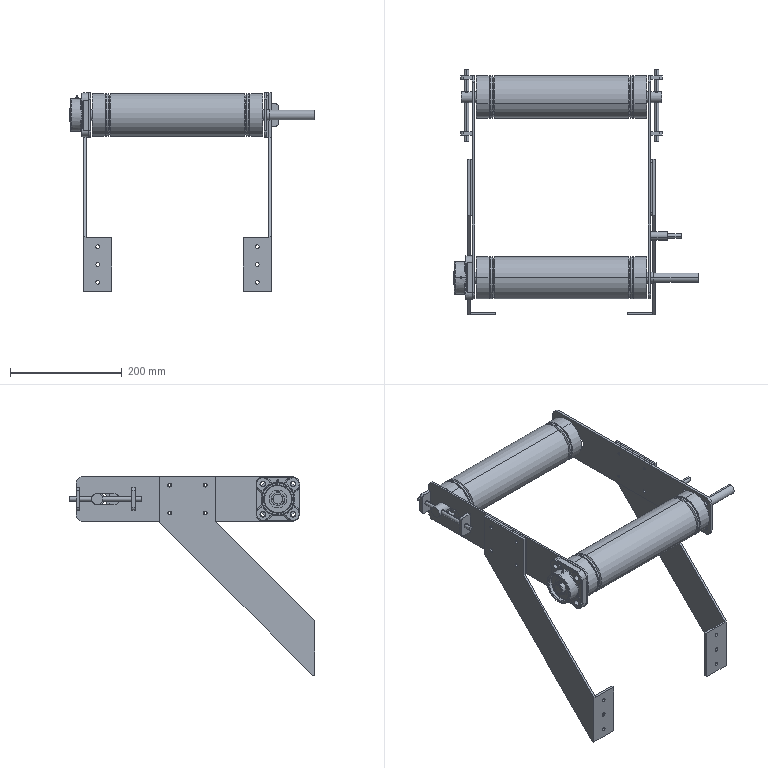Assembly | SolidWorks | mm | 19 component files | 25 solids | 709 faces | box 439 x 439.86 x 356 mm | volume 1830809 mm3 | cylinder 284 | plane 170 | torus 100 | spline 59 | sphere 52 | cone 44 | commonest cylinder face diameters 5 x32 2 x30 7 x28 76 x20 8.5 x16 10 x16 24 x14 20 x14
Bill of materials:
YL1.sldasm-Part-70 | 2 |  | Thin, flat rectangular plate. Two corners on one long edge are rounded and the opposite two are square. It has four small through-holes in a rectangular pattern.
YL1.sldasm-Part-85 | 2 |  | Small, thick rectangular block or plate with one central round through-hole. The two corners on one short side are rounded.
YL1.sldasm-Part-87 | 2 |  | Small, thick rectangular block or plate with one central round through-hole. The two corners on one short side are rounded.
YL1.sldasm-Part-90 | 2 |  | Long, thin, flat strip plate with rounded corners. Near one end it has a large round hole with four small holes around it. Four smaller holes sit in a rectangular pattern near mid-length, and there is an elongated slot near the other end.
BeltLineSupportPlate | 1 |  | Bent sheet-like bracket. A diagonal strip joins a rectangular tab at each end; the two tabs lie in different planes. One end tab has three holes in a line and the other has four holes in a square pattern.
deep groove ball bearings gb | 2 |  | Ring-shaped part that looks like a ball bearing: concentric inner and outer rings with a ring of spherical balls between them, and an open bore.
DrivenRoller | 1 |  | Hollow cylindrical sleeve or tube with a thick wall. Near each end, the outer surface has a pair of narrow circumferential grooves.
DrivenShaft | 1 |  | Long, slender solid cylindrical rod or shaft. It has one radial cross-hole near each end, and faint lines next to the end segments suggest small steps or seams.
DriveRoller | 1 |  | Bent sheet-like bracket. A diagonal strip joins a rectangular tab at each end; the two tabs lie in different planes. One end tab has three holes in a line and the other has four holes in a square pattern.
LeadScrewM8x130 | 2 |  | Large-diameter cylindrical body with a pair of circumferential grooves near each end. A stepped, smaller-diameter shaft sticks out coaxially from each end face.
MirrorBeltLineSupportPlate | 1 |  | Plain solid cylindrical rod with flat ends and no visible features.
SquarePillowBlockBearingUCFU203 | 1 |  | Flanged housing: a square flange with rounded corners and four through-holes, a cylindrical boss on one side, and a central bore with a raised inner ring. A small nipple-like protrusion is on the boss's outer surface, and a small hex-shaped feature is visible on its side.
TorqueArmMountingShaft-1 | 1 |  | Solid stepped cylindrical shaft/pin with two coaxial round sections: a larger-diameter body and a smaller-diameter, slightly shorter spigot. The step between them is a flat, square shoulder, and both ends are flat.
Mates:
1. concentric | DrivenRoller-1 face at (7087.506, 3057.679, 47.375) dir (1, 0, 0) r 23.5 | deep groove ball bearings gb-2 face at (5788.035, 3057.679, 47.375) dir (-1, 0, 0) r 5
2. concentric | deep groove ball bearings gb-1 face at (6083.717, 3057.679, 47.375) dir (1, 0, 0) r 13 | DrivenRoller-1 face at (10398.381, 3057.679, 47.375) dir (1, 0, 0) r 34
3. coincident | DrivenRoller-1 face at (6071.006, 3074.243, 53.023) dir (1, 0, 0) | deep groove ball bearings gb-1 face at (6071.006, 3061.43, 59.822) dir (-1, 0, 0)
4. coincident | DrivenRoller-1 face at (5799.006, 3079.922, 54.96) dir (-1, 0, 0) | deep groove ball bearings gb-2 face at (5799.006, 3063.772, 35.891) dir (1, 0, 0)
5. concentric | deep groove ball bearings gb-1 face at (6083.717, 3057.679, 47.375) dir (1, 0, 0) r 13 | DrivenShaft-1 face at (6115.006, 3057.679, 47.375) dir (1, 0, 0) r 10
6. coincident | BeltLineSidePlate-1/YL1.sldasm-Part-70-1 face at (6099.006, 2845.679, 87.375) dir (0, 0, 1) | BeltLineSupportPlate-1 face at (6099.006, 2945.997, 87.375) dir (0, 0, 1)
7. coincident | BeltLineSidePlate-1/YL1.sldasm-Part-70-1 face at (6099.006, 2845.679, 6.964) dir (1, 0, 0) | BeltLineSupportPlate-1 face at (6099.006, 2625.997, -268.625) dir (-1, 0, 0)
8. concentric | BeltLineSidePlate-1/YL1.sldasm-Part-70-1 face at (6099.006, 2927.997, 72.375) dir (1, 0, 0) r 2.5 | BeltLineSupportPlate-1 face at (6099.006, 2927.997, 72.375) dir (-1, 0, 0) r 3.5
9. coincident | BeltLineSidePlate-1/YL1.sldasm-Part-90-1 face at (6095.006, 4695.679, 85.375) dir (1, 0, 0) | TorqueArmMountingShaft-1-1 face at (6095.006, 2808.679, 47.375) dir (-1, 0, 0)
10. concentric | deep groove ball bearings gb-1 face at (6083.717, 3057.679, 47.375) dir (1, 0, 0) r 13 | BeltLineSidePlate-3/YL1.sldasm-Part-90-1 face at (4375.006, 3057.679, 47.375) dir (1, 0, 0) r 10
11. coincident | DrivenRoller-1 face at (5782.506, 3093.646, 59.64) dir (-1, 0, 0) | DriveRoller-1 face at (5782.506, 2771.679, 47.375) dir (-1, 0, 0)
12. concentric | DrivenShaft-1 face at (5764.506, 3067.679, 47.375) dir (0, 1, 0) r 4.5 | LeadScrewM8x130-3 face at (5764.506, 3007.679, 47.375) dir (0, 1, 0) r 4
13. distance | BeltLineSidePlate-3/YL1.sldasm-Part-90-1 face at (5779.006, 4695.679, 84.375) dir (1, 0, 0) | DriveRoller-1 face at (5782.506, 2771.679, 47.375) dir (-1, 0, 0)
14. concentric | SquarePillowBlockBearingUCFU203-3 face at (5764.606, 2760.679, 74.375) dir (1, 0, 0) r 5.25 | BeltLineSidePlate-3/YL1.sldasm-Part-90-1 face at (5775.006, 2760.679, 74.375) dir (-1, 0, 0) r 4.25
15. concentric | SquarePillowBlockBearingUCFU203-3 face at (5743.006, 2733.679, 47.375) dir (-1, 0, 0) r 29.5 | DriveRoller-1 face at (5741.506, 2733.679, 47.375) dir (-1, 0, 0) r 8.5
16. concentric | DriveRoller-1 face at (5741.506, 2733.679, 47.375) dir (-1, 0, 0) r 8.5 | BeltLineSidePlate-3/YL1.sldasm-Part-90-1 face at (5820.506, 2733.679, 47.375) dir (-1, 0, 0) r 13.5
17. coincident | SquarePillowBlockBearingUCFU203-3 face at (5775.006, 2706.679, 74.375) dir (1, 0, 0) | BeltLineSidePlate-3/YL1.sldasm-Part-90-1 face at (5775.006, 4695.679, 9.375) dir (-1, 0, 0)